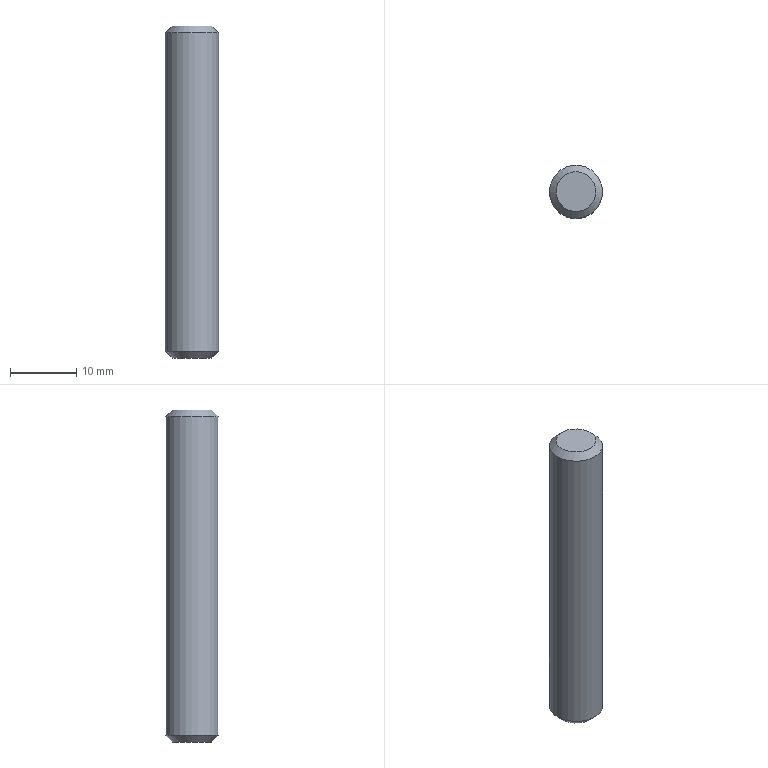Component | NX | PIN | 1 solid | 5 faces | box 8 x 8 x 50 mm | volume 2490 mm3 | plane 2 | cone 2 | cylinder 1 | commonest cylinder face diameters 8 x1
STEP:
#1=CARTESIAN_POINT('',(0.,0.,0.));
#2=DIRECTION('',(0.,0.,1.));
#3=DIRECTION('',(1.,0.,0.));
#4=AXIS2_PLACEMENT_3D('',#1,#2,#3);
#5=CARTESIAN_POINT('',(27.25,-42.002,114.));
#6=VERTEX_POINT('',#5);
#7=CARTESIAN_POINT('',(24.25,-42.002,114.));
#8=DIRECTION('',(0.,0.,1.));
#9=DIRECTION('',(1.,0.,0.));
#10=AXIS2_PLACEMENT_3D('',#7,#8,#9);
#11=CIRCLE('',#10,3.);
#12=CARTESIAN_POINT('',(24.25,-42.002,114.));
#13=DIRECTION('',(0.,0.,1.));
#14=DIRECTION('',(1.,0.,0.));
#15=AXIS2_PLACEMENT_3D('',#12,#13,#14);
#16=PLANE('',#15);
#17=CARTESIAN_POINT('',(0.,0.));
#18=DIRECTION('',(1.,0.));
#19=AXIS2_PLACEMENT_2D('',#17,#18);
#20=CIRCLE('',#19,3.);
#21=(GEOMETRIC_REPRESENTATION_CONTEXT(2)PARAMETRIC_REPRESENTATION_CONTEXT()REPRESENTATION_CONTEXT('',''));
#22=DEFINITIONAL_REPRESENTATION('',(#20),#21);
#23=PCURVE('',#16,#22);
#24=CARTESIAN_POINT('',(24.25,-42.002,113.));
#25=DIRECTION('',(0.,0.,-1.));
#26=DIRECTION('',(-1.,0.,0.));
#27=AXIS2_PLACEMENT_3D('',#24,#25,#26);
#28=CONICAL_SURFACE('',#27,4.,0.7854);
#29=CARTESIAN_POINT('',(9.425,-1.));
#30=DIRECTION('',(-1.,0.));
#31=VECTOR('',#30,1.);
#32=LINE('',#29,#31);
#33=(GEOMETRIC_REPRESENTATION_CONTEXT(2)PARAMETRIC_REPRESENTATION_CONTEXT()REPRESENTATION_CONTEXT('',''));
#34=DEFINITIONAL_REPRESENTATION('',(#32),#33);
#35=PCURVE('',#28,#34);
#36=SURFACE_CURVE('',#11,(#23,#35),.PCURVE_S1.);
#37=EDGE_CURVE('',#6,#6,#36,.T.);
#38=ORIENTED_EDGE('',*,*,#37,.T.);
#39=EDGE_LOOP('',(#38));
#40=FACE_BOUND('',#39,.T.);
#41=ADVANCED_FACE('',(#40),#16,.T.);
#42=CARTESIAN_POINT('',(21.25,-42.002,64.));
#43=VERTEX_POINT('',#42);
#44=CARTESIAN_POINT('',(24.25,-42.002,64.));
#45=DIRECTION('',(0.,0.,-1.));
#46=DIRECTION('',(-1.,0.,0.));
#47=AXIS2_PLACEMENT_3D('',#44,#45,#46);
#48=CIRCLE('',#47,3.);
#49=CARTESIAN_POINT('',(24.25,-42.002,64.));
#50=DIRECTION('',(0.,0.,-1.));
#51=DIRECTION('',(-1.,0.,0.));
#52=AXIS2_PLACEMENT_3D('',#49,#50,#51);
#53=PLANE('',#52);
#54=CARTESIAN_POINT('',(0.,0.));
#55=DIRECTION('',(1.,0.));
#56=AXIS2_PLACEMENT_2D('',#54,#55);
#57=CIRCLE('',#56,3.);
#58=(GEOMETRIC_REPRESENTATION_CONTEXT(2)PARAMETRIC_REPRESENTATION_CONTEXT()REPRESENTATION_CONTEXT('',''));
#59=DEFINITIONAL_REPRESENTATION('',(#57),#58);
#60=PCURVE('',#53,#59);
#61=CARTESIAN_POINT('',(24.25,-42.002,65.));
#62=DIRECTION('',(0.,0.,1.));
#63=DIRECTION('',(1.,0.,0.));
#64=AXIS2_PLACEMENT_3D('',#61,#62,#63);
#65=CONICAL_SURFACE('',#64,4.,0.7854);
#66=CARTESIAN_POINT('',(9.425,-1.));
#67=DIRECTION('',(-1.,0.));
#68=VECTOR('',#67,1.);
#69=LINE('',#66,#68);
#70=(GEOMETRIC_REPRESENTATION_CONTEXT(2)PARAMETRIC_REPRESENTATION_CONTEXT()REPRESENTATION_CONTEXT('',''));
#71=DEFINITIONAL_REPRESENTATION('',(#69),#70);
#72=PCURVE('',#65,#71);
#73=SURFACE_CURVE('',#48,(#60,#72),.PCURVE_S1.);
#74=EDGE_CURVE('',#43,#43,#73,.T.);
#75=ORIENTED_EDGE('',*,*,#74,.T.);
#76=EDGE_LOOP('',(#75));
#77=FACE_BOUND('',#76,.T.);
#78=ADVANCED_FACE('',(#77),#53,.T.);
#79=CARTESIAN_POINT('',(20.25,-42.002,65.));
#80=VERTEX_POINT('',#79);
#81=CARTESIAN_POINT('',(28.25,-42.002,65.));
#82=VERTEX_POINT('',#81);
#83=CARTESIAN_POINT('',(24.25,-42.002,65.));
#84=DIRECTION('',(0.,0.,1.));
#85=DIRECTION('',(-1.,0.,0.));
#86=AXIS2_PLACEMENT_3D('',#83,#84,#85);
#87=CIRCLE('',#86,4.);
#88=CARTESIAN_POINT('',(24.25,-42.002,64.));
#89=DIRECTION('',(0.,0.,1.));
#90=DIRECTION('',(1.,0.,0.));
#91=AXIS2_PLACEMENT_3D('',#88,#89,#90);
#92=CYLINDRICAL_SURFACE('',#91,4.);
#93=CARTESIAN_POINT('',(3.142,1.));
#94=DIRECTION('',(1.,0.));
#95=VECTOR('',#94,1.);
#96=LINE('',#93,#95);
#97=(GEOMETRIC_REPRESENTATION_CONTEXT(2)PARAMETRIC_REPRESENTATION_CONTEXT()REPRESENTATION_CONTEXT('',''));
#98=DEFINITIONAL_REPRESENTATION('',(#96),#97);
#99=PCURVE('',#92,#98);
#100=CARTESIAN_POINT('',(3.142,0.));
#101=DIRECTION('',(1.,0.));
#102=VECTOR('',#101,1.);
#103=LINE('',#100,#102);
#104=(GEOMETRIC_REPRESENTATION_CONTEXT(2)PARAMETRIC_REPRESENTATION_CONTEXT()REPRESENTATION_CONTEXT('',''));
#105=DEFINITIONAL_REPRESENTATION('',(#103),#104);
#106=PCURVE('',#65,#105);
#107=SURFACE_CURVE('',#87,(#99,#106),.PCURVE_S1.);
#108=EDGE_CURVE('',#80,#82,#107,.T.);
#109=ORIENTED_EDGE('',*,*,#108,.T.);
#110=CARTESIAN_POINT('',(28.25,-42.002,113.));
#111=VERTEX_POINT('',#110);
#112=CARTESIAN_POINT('',(28.25,-42.002,65.));
#113=CARTESIAN_POINT('',(28.25,-42.002,113.));
#114=B_SPLINE_CURVE_WITH_KNOTS('',1,(#112,#113),.UNSPECIFIED.,.F.,.F.,(2,2),(1.,49.),.PIECEWISE_BEZIER_KNOTS.);
#115=CARTESIAN_POINT('',(6.283,0.));
#116=DIRECTION('',(0.,1.));
#117=VECTOR('',#116,1.);
#118=LINE('',#115,#117);
#119=(GEOMETRIC_REPRESENTATION_CONTEXT(2)PARAMETRIC_REPRESENTATION_CONTEXT()REPRESENTATION_CONTEXT('',''));
#120=DEFINITIONAL_REPRESENTATION('',(#118),#119);
#121=PCURVE('',#92,#120);
#122=CARTESIAN_POINT('',(0.,0.));
#123=DIRECTION('',(0.,1.));
#124=VECTOR('',#123,1.);
#125=LINE('',#122,#124);
#126=(GEOMETRIC_REPRESENTATION_CONTEXT(2)PARAMETRIC_REPRESENTATION_CONTEXT()REPRESENTATION_CONTEXT('',''));
#127=DEFINITIONAL_REPRESENTATION('',(#125),#126);
#128=PCURVE('',#92,#127);
#129=SEAM_CURVE('',#114,(#121,#128),.PCURVE_S1.);
#130=EDGE_CURVE('',#82,#111,#129,.T.);
#131=ORIENTED_EDGE('',*,*,#130,.T.);
#132=CARTESIAN_POINT('',(24.25,-42.002,113.));
#133=DIRECTION('',(0.,0.,-1.));
#134=DIRECTION('',(1.,0.,0.));
#135=AXIS2_PLACEMENT_3D('',#132,#133,#134);
#136=CIRCLE('',#135,4.);
#137=CARTESIAN_POINT('',(6.283,49.));
#138=DIRECTION('',(-1.,0.));
#139=VECTOR('',#138,1.);
#140=LINE('',#137,#139);
#141=(GEOMETRIC_REPRESENTATION_CONTEXT(2)PARAMETRIC_REPRESENTATION_CONTEXT()REPRESENTATION_CONTEXT('',''));
#142=DEFINITIONAL_REPRESENTATION('',(#140),#141);
#143=PCURVE('',#92,#142);
#144=CARTESIAN_POINT('',(3.142,0.));
#145=DIRECTION('',(1.,0.));
#146=VECTOR('',#145,1.);
#147=LINE('',#144,#146);
#148=(GEOMETRIC_REPRESENTATION_CONTEXT(2)PARAMETRIC_REPRESENTATION_CONTEXT()REPRESENTATION_CONTEXT('',''));
#149=DEFINITIONAL_REPRESENTATION('',(#147),#148);
#150=PCURVE('',#28,#149);
#151=SURFACE_CURVE('',#136,(#143,#150),.PCURVE_S1.);
#152=EDGE_CURVE('',#111,#111,#151,.T.);
#153=ORIENTED_EDGE('',*,*,#152,.T.);
#154=ORIENTED_EDGE('',*,*,#130,.F.);
#155=CARTESIAN_POINT('',(24.25,-42.002,65.));
#156=DIRECTION('',(0.,0.,1.));
#157=DIRECTION('',(-1.,0.,0.));
#158=AXIS2_PLACEMENT_3D('',#155,#156,#157);
#159=CIRCLE('',#158,4.);
#160=CARTESIAN_POINT('',(-3.142,1.));
#161=DIRECTION('',(1.,0.));
#162=VECTOR('',#161,1.);
#163=LINE('',#160,#162);
#164=(GEOMETRIC_REPRESENTATION_CONTEXT(2)PARAMETRIC_REPRESENTATION_CONTEXT()REPRESENTATION_CONTEXT('',''));
#165=DEFINITIONAL_REPRESENTATION('',(#163),#164);
#166=PCURVE('',#92,#165);
#167=CARTESIAN_POINT('',(3.142,0.));
#168=DIRECTION('',(1.,0.));
#169=VECTOR('',#168,1.);
#170=LINE('',#167,#169);
#171=(GEOMETRIC_REPRESENTATION_CONTEXT(2)PARAMETRIC_REPRESENTATION_CONTEXT()REPRESENTATION_CONTEXT('',''));
#172=DEFINITIONAL_REPRESENTATION('',(#170),#171);
#173=PCURVE('',#65,#172);
#174=SURFACE_CURVE('',#159,(#166,#173),.PCURVE_S1.);
#175=EDGE_CURVE('',#82,#80,#174,.T.);
#176=ORIENTED_EDGE('',*,*,#175,.T.);
#177=EDGE_LOOP('',(#109,#131,#153,#154,#176));
#178=FACE_BOUND('',#177,.T.);
#179=ADVANCED_FACE('',(#178),#92,.T.);
#180=ORIENTED_EDGE('',*,*,#74,.F.);
#181=CARTESIAN_POINT('',(21.25,-42.002,64.));
#182=CARTESIAN_POINT('',(20.25,-42.002,65.));
#183=B_SPLINE_CURVE_WITH_KNOTS('',1,(#181,#182),.UNSPECIFIED.,.F.,.F.,(2,2),(-1.414,0.),.PIECEWISE_BEZIER_KNOTS.);
#184=CARTESIAN_POINT('',(9.425,0.));
#185=DIRECTION('',(0.,1.));
#186=VECTOR('',#185,1.);
#187=LINE('',#184,#186);
#188=(GEOMETRIC_REPRESENTATION_CONTEXT(2)PARAMETRIC_REPRESENTATION_CONTEXT()REPRESENTATION_CONTEXT('',''));
#189=DEFINITIONAL_REPRESENTATION('',(#187),#188);
#190=PCURVE('',#65,#189);
#191=CARTESIAN_POINT('',(3.142,0.));
#192=DIRECTION('',(0.,1.));
#193=VECTOR('',#192,1.);
#194=LINE('',#191,#193);
#195=(GEOMETRIC_REPRESENTATION_CONTEXT(2)PARAMETRIC_REPRESENTATION_CONTEXT()REPRESENTATION_CONTEXT('',''));
#196=DEFINITIONAL_REPRESENTATION('',(#194),#195);
#197=PCURVE('',#65,#196);
#198=SEAM_CURVE('',#183,(#190,#197),.PCURVE_S1.);
#199=EDGE_CURVE('',#43,#80,#198,.T.);
#200=ORIENTED_EDGE('',*,*,#199,.T.);
#201=ORIENTED_EDGE('',*,*,#175,.F.);
#202=ORIENTED_EDGE('',*,*,#108,.F.);
#203=ORIENTED_EDGE('',*,*,#199,.F.);
#204=EDGE_LOOP('',(#180,#200,#201,#202,#203));
#205=FACE_BOUND('',#204,.T.);
#206=ADVANCED_FACE('',(#205),#65,.T.);
#207=ORIENTED_EDGE('',*,*,#37,.F.);
#208=CARTESIAN_POINT('',(27.25,-42.002,114.));
#209=CARTESIAN_POINT('',(28.25,-42.002,113.));
#210=B_SPLINE_CURVE_WITH_KNOTS('',1,(#208,#209),.UNSPECIFIED.,.F.,.F.,(2,2),(-1.414,0.),.PIECEWISE_BEZIER_KNOTS.);
#211=CARTESIAN_POINT('',(9.425,0.));
#212=DIRECTION('',(0.,1.));
#213=VECTOR('',#212,1.);
#214=LINE('',#211,#213);
#215=(GEOMETRIC_REPRESENTATION_CONTEXT(2)PARAMETRIC_REPRESENTATION_CONTEXT()REPRESENTATION_CONTEXT('',''));
#216=DEFINITIONAL_REPRESENTATION('',(#214),#215);
#217=PCURVE('',#28,#216);
#218=CARTESIAN_POINT('',(3.142,0.));
#219=DIRECTION('',(0.,1.));
#220=VECTOR('',#219,1.);
#221=LINE('',#218,#220);
#222=(GEOMETRIC_REPRESENTATION_CONTEXT(2)PARAMETRIC_REPRESENTATION_CONTEXT()REPRESENTATION_CONTEXT('',''));
#223=DEFINITIONAL_REPRESENTATION('',(#221),#222);
#224=PCURVE('',#28,#223);
#225=SEAM_CURVE('',#210,(#217,#224),.PCURVE_S1.);
#226=EDGE_CURVE('',#6,#111,#225,.T.);
#227=ORIENTED_EDGE('',*,*,#226,.T.);
#228=ORIENTED_EDGE('',*,*,#152,.F.);
#229=ORIENTED_EDGE('',*,*,#226,.F.);
#230=EDGE_LOOP('',(#207,#227,#228,#229));
#231=FACE_BOUND('',#230,.T.);
#232=ADVANCED_FACE('',(#231),#28,.T.);
#233=CLOSED_SHELL('',(#41,#78,#179,#206,#232));
#234=MANIFOLD_SOLID_BREP('',#233);
#235=(LENGTH_UNIT()NAMED_UNIT(*)SI_UNIT(.MILLI.,.METRE.));
#236=UNCERTAINTY_MEASURE_WITH_UNIT(LENGTH_MEASURE(0.00001),#235,'','');
#237=(NAMED_UNIT(*)PLANE_ANGLE_UNIT()SI_UNIT($,.RADIAN.));
#238=(NAMED_UNIT(*)SI_UNIT($,.STERADIAN.)SOLID_ANGLE_UNIT());
#239=(GEOMETRIC_REPRESENTATION_CONTEXT(3)GLOBAL_UNCERTAINTY_ASSIGNED_CONTEXT((#236))GLOBAL_UNIT_ASSIGNED_CONTEXT((#235,#237,#238))REPRESENTATION_CONTEXT('',''));
#240=ADVANCED_BREP_SHAPE_REPRESENTATION('',(#4,#234),#239);